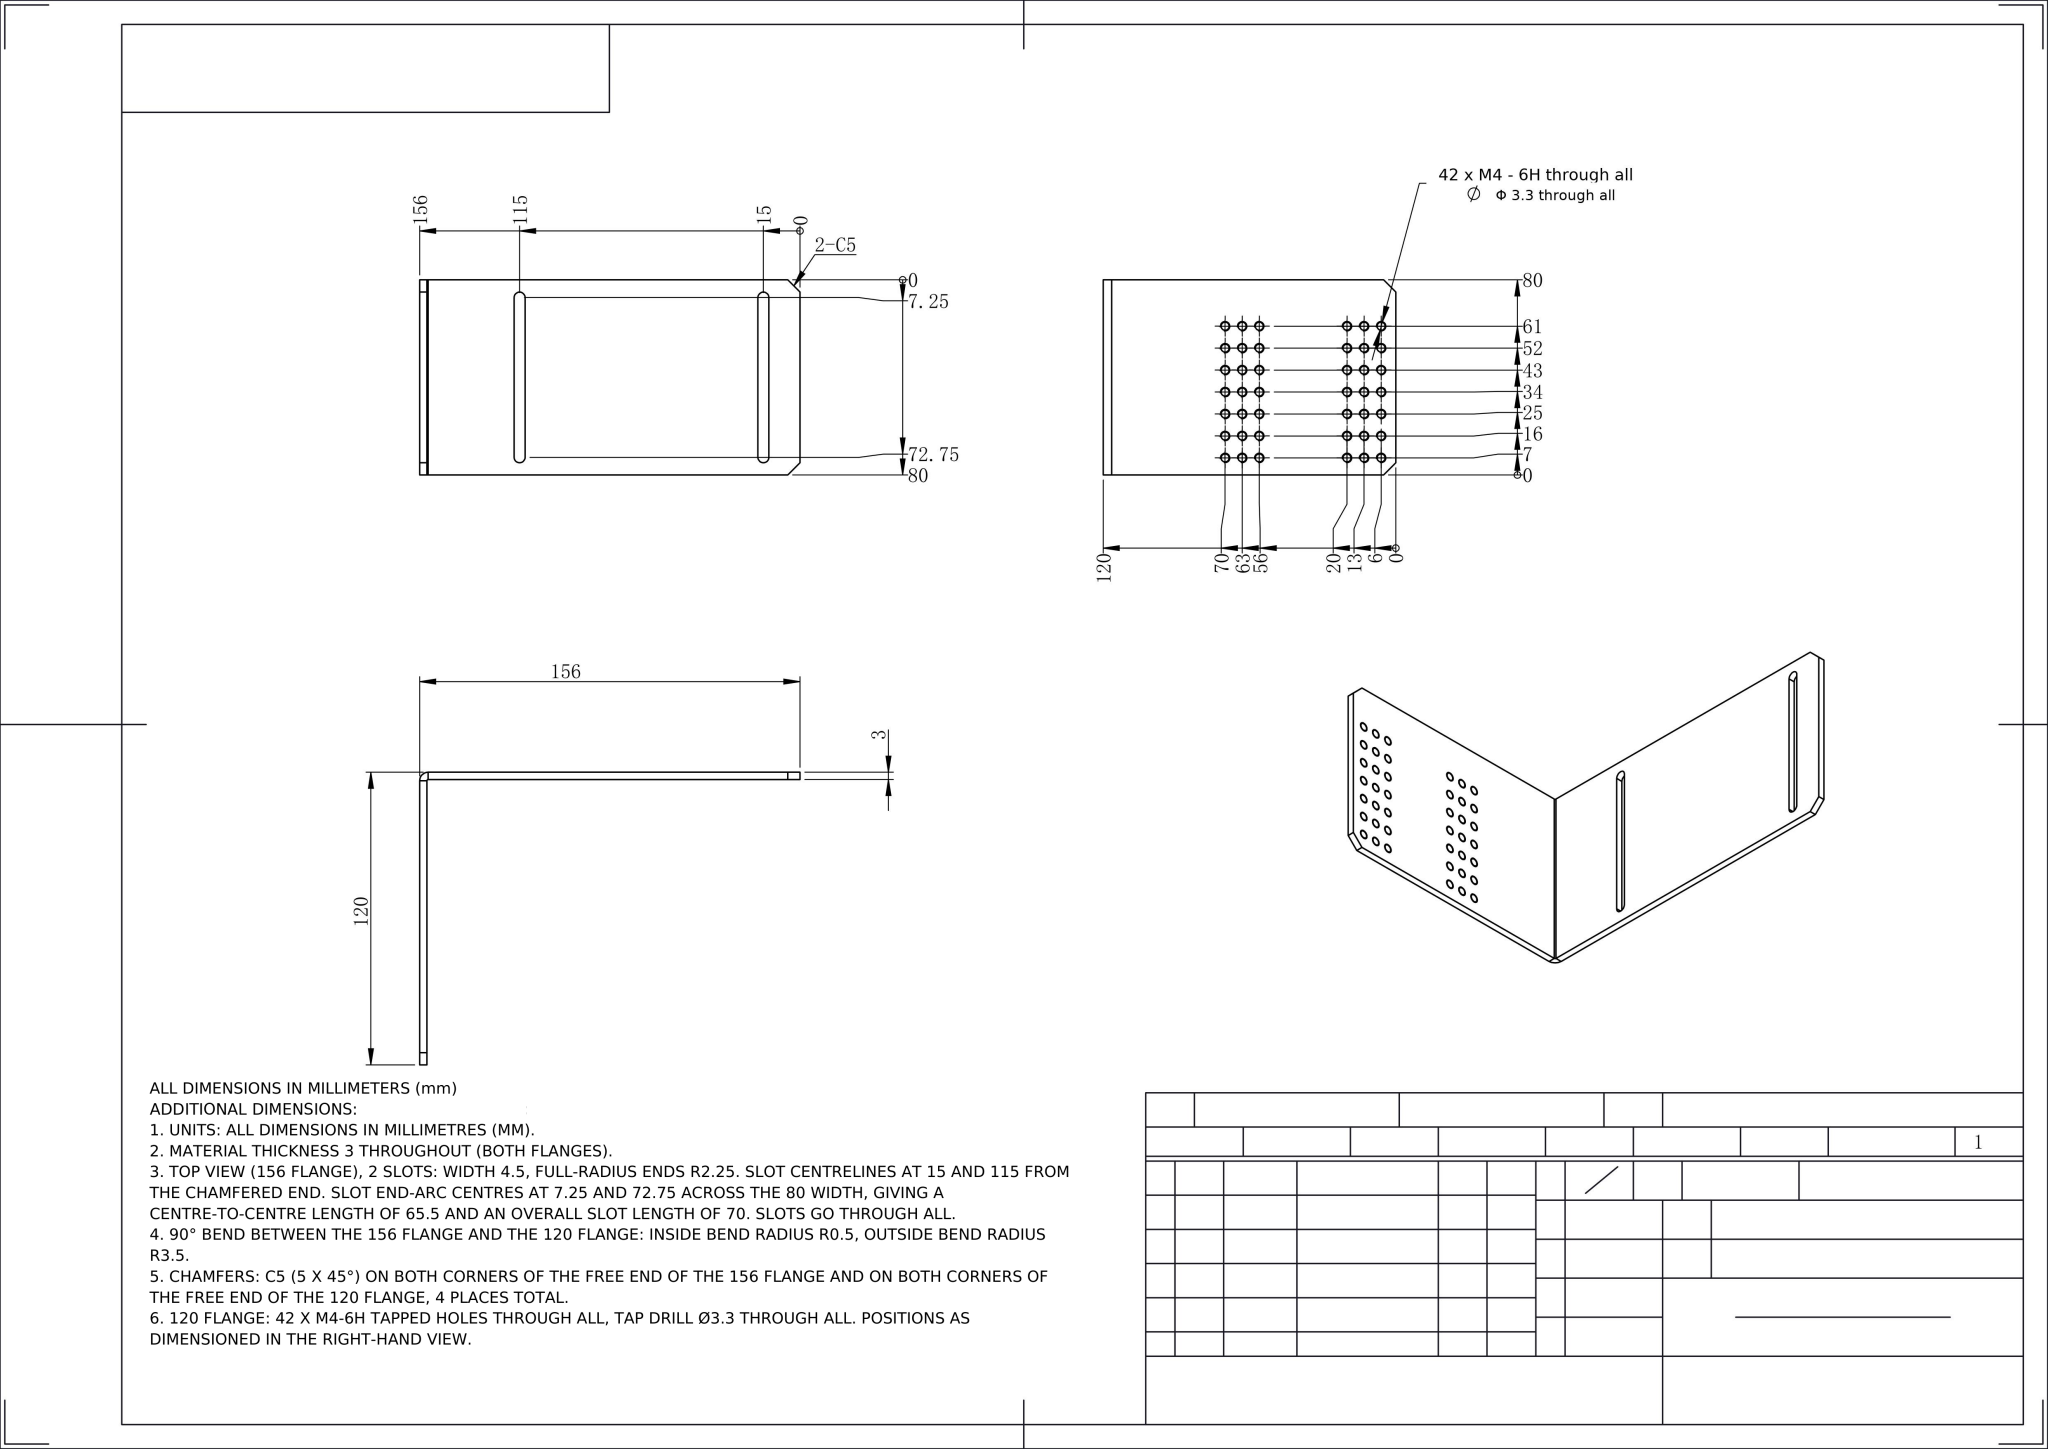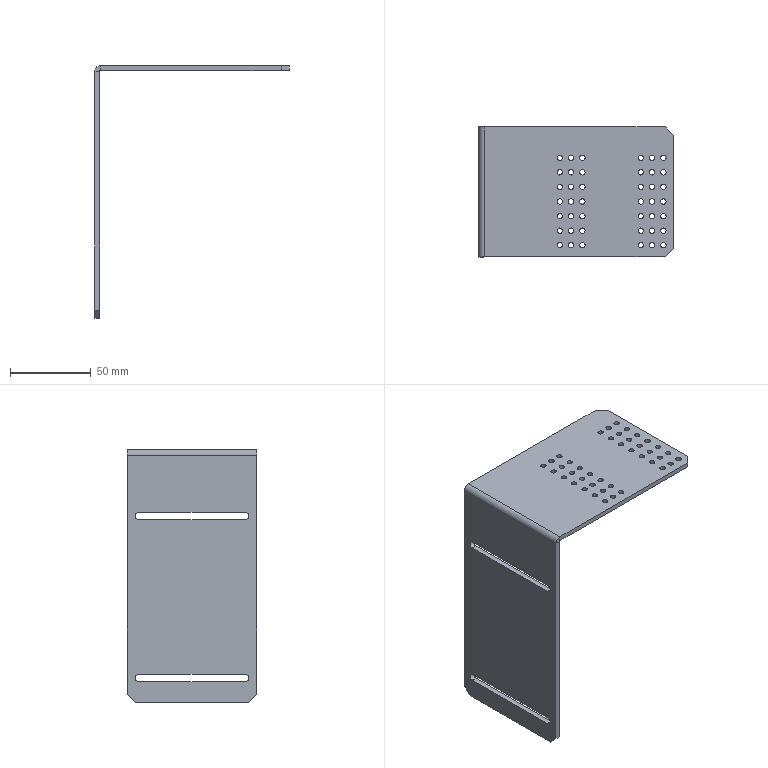Part | NX | mm | Perforated U-Channel Shelf Bracket 156mm | 1 solid | 110 faces | box 120 x 80 x 156 mm | volume 62222 mm3 | cylinder 90 | plane 20 | commonest cylinder face diameters 3.3 x84 4.5 x4 7 x1 1 x1